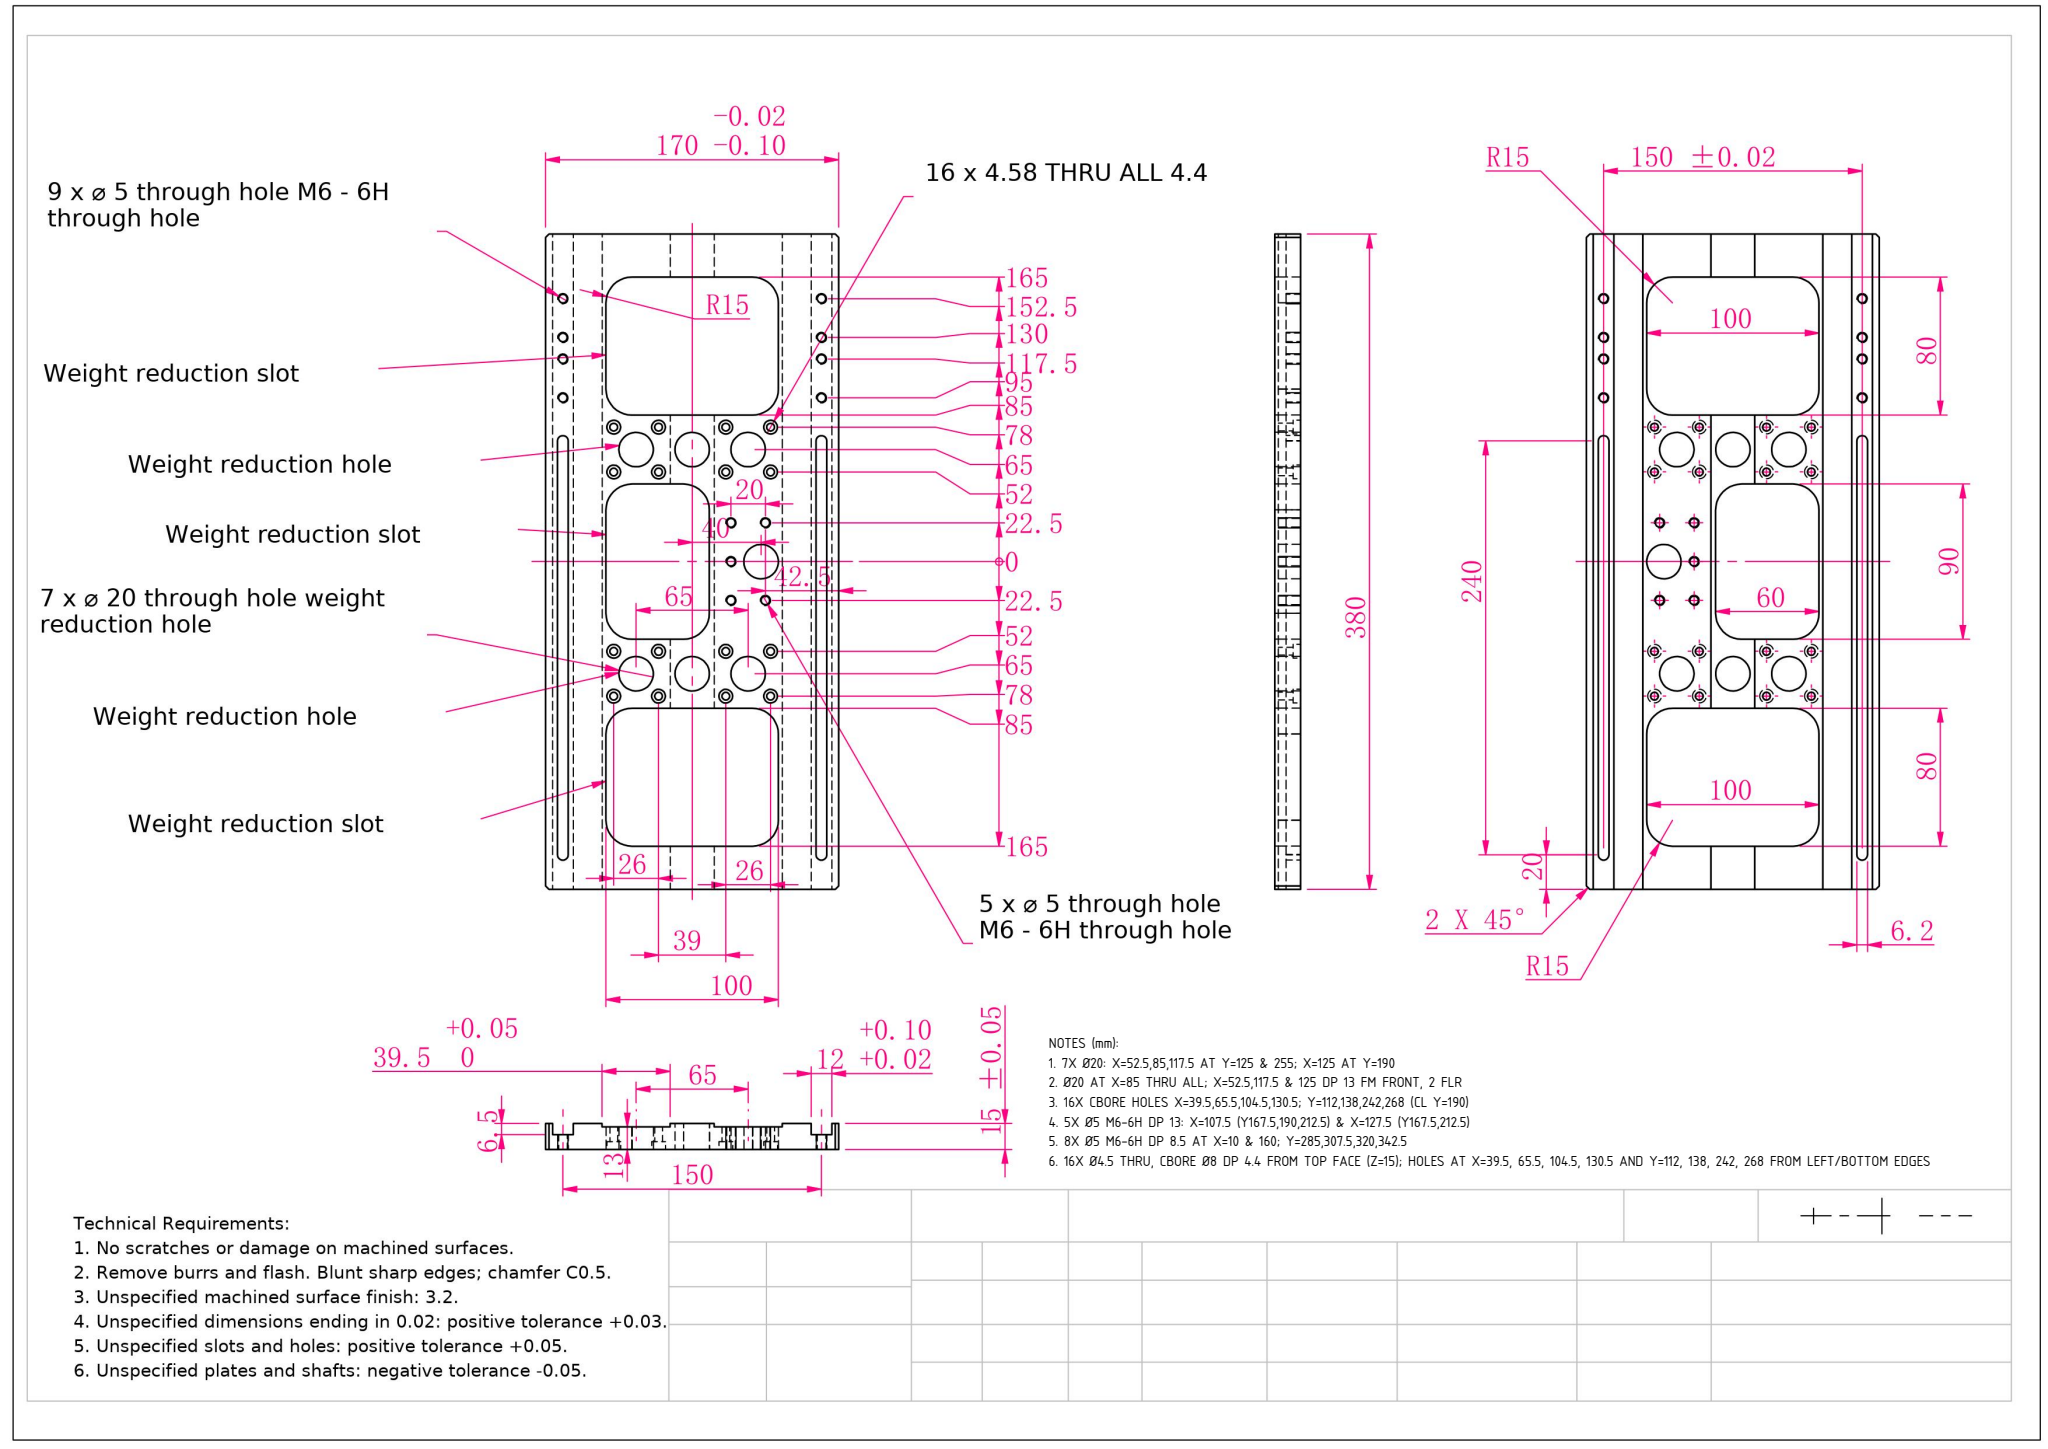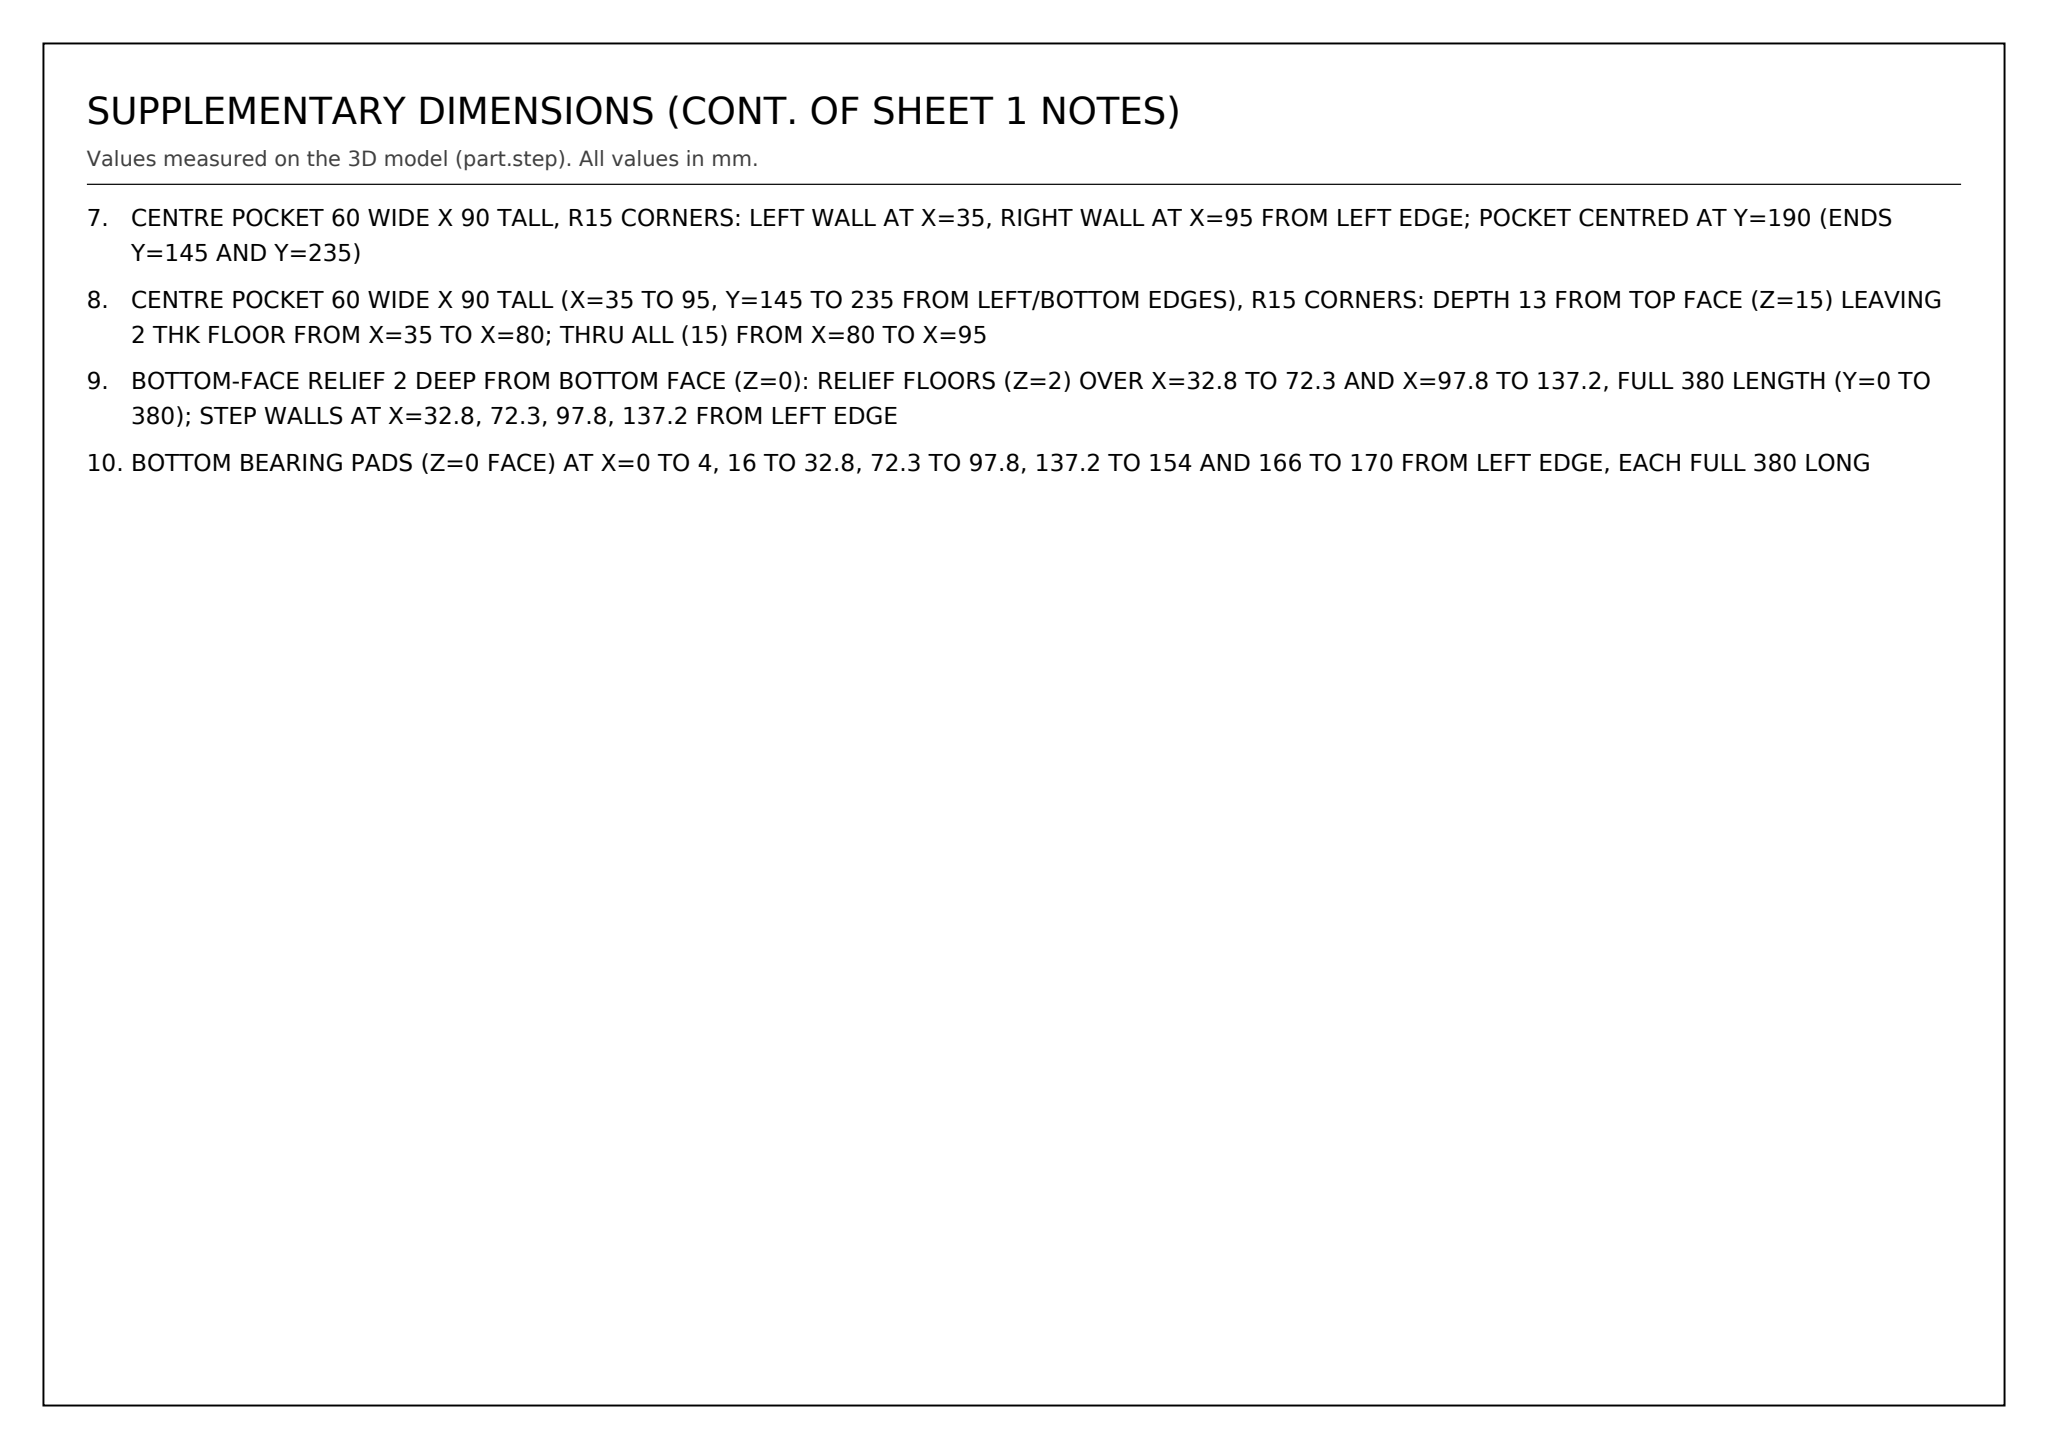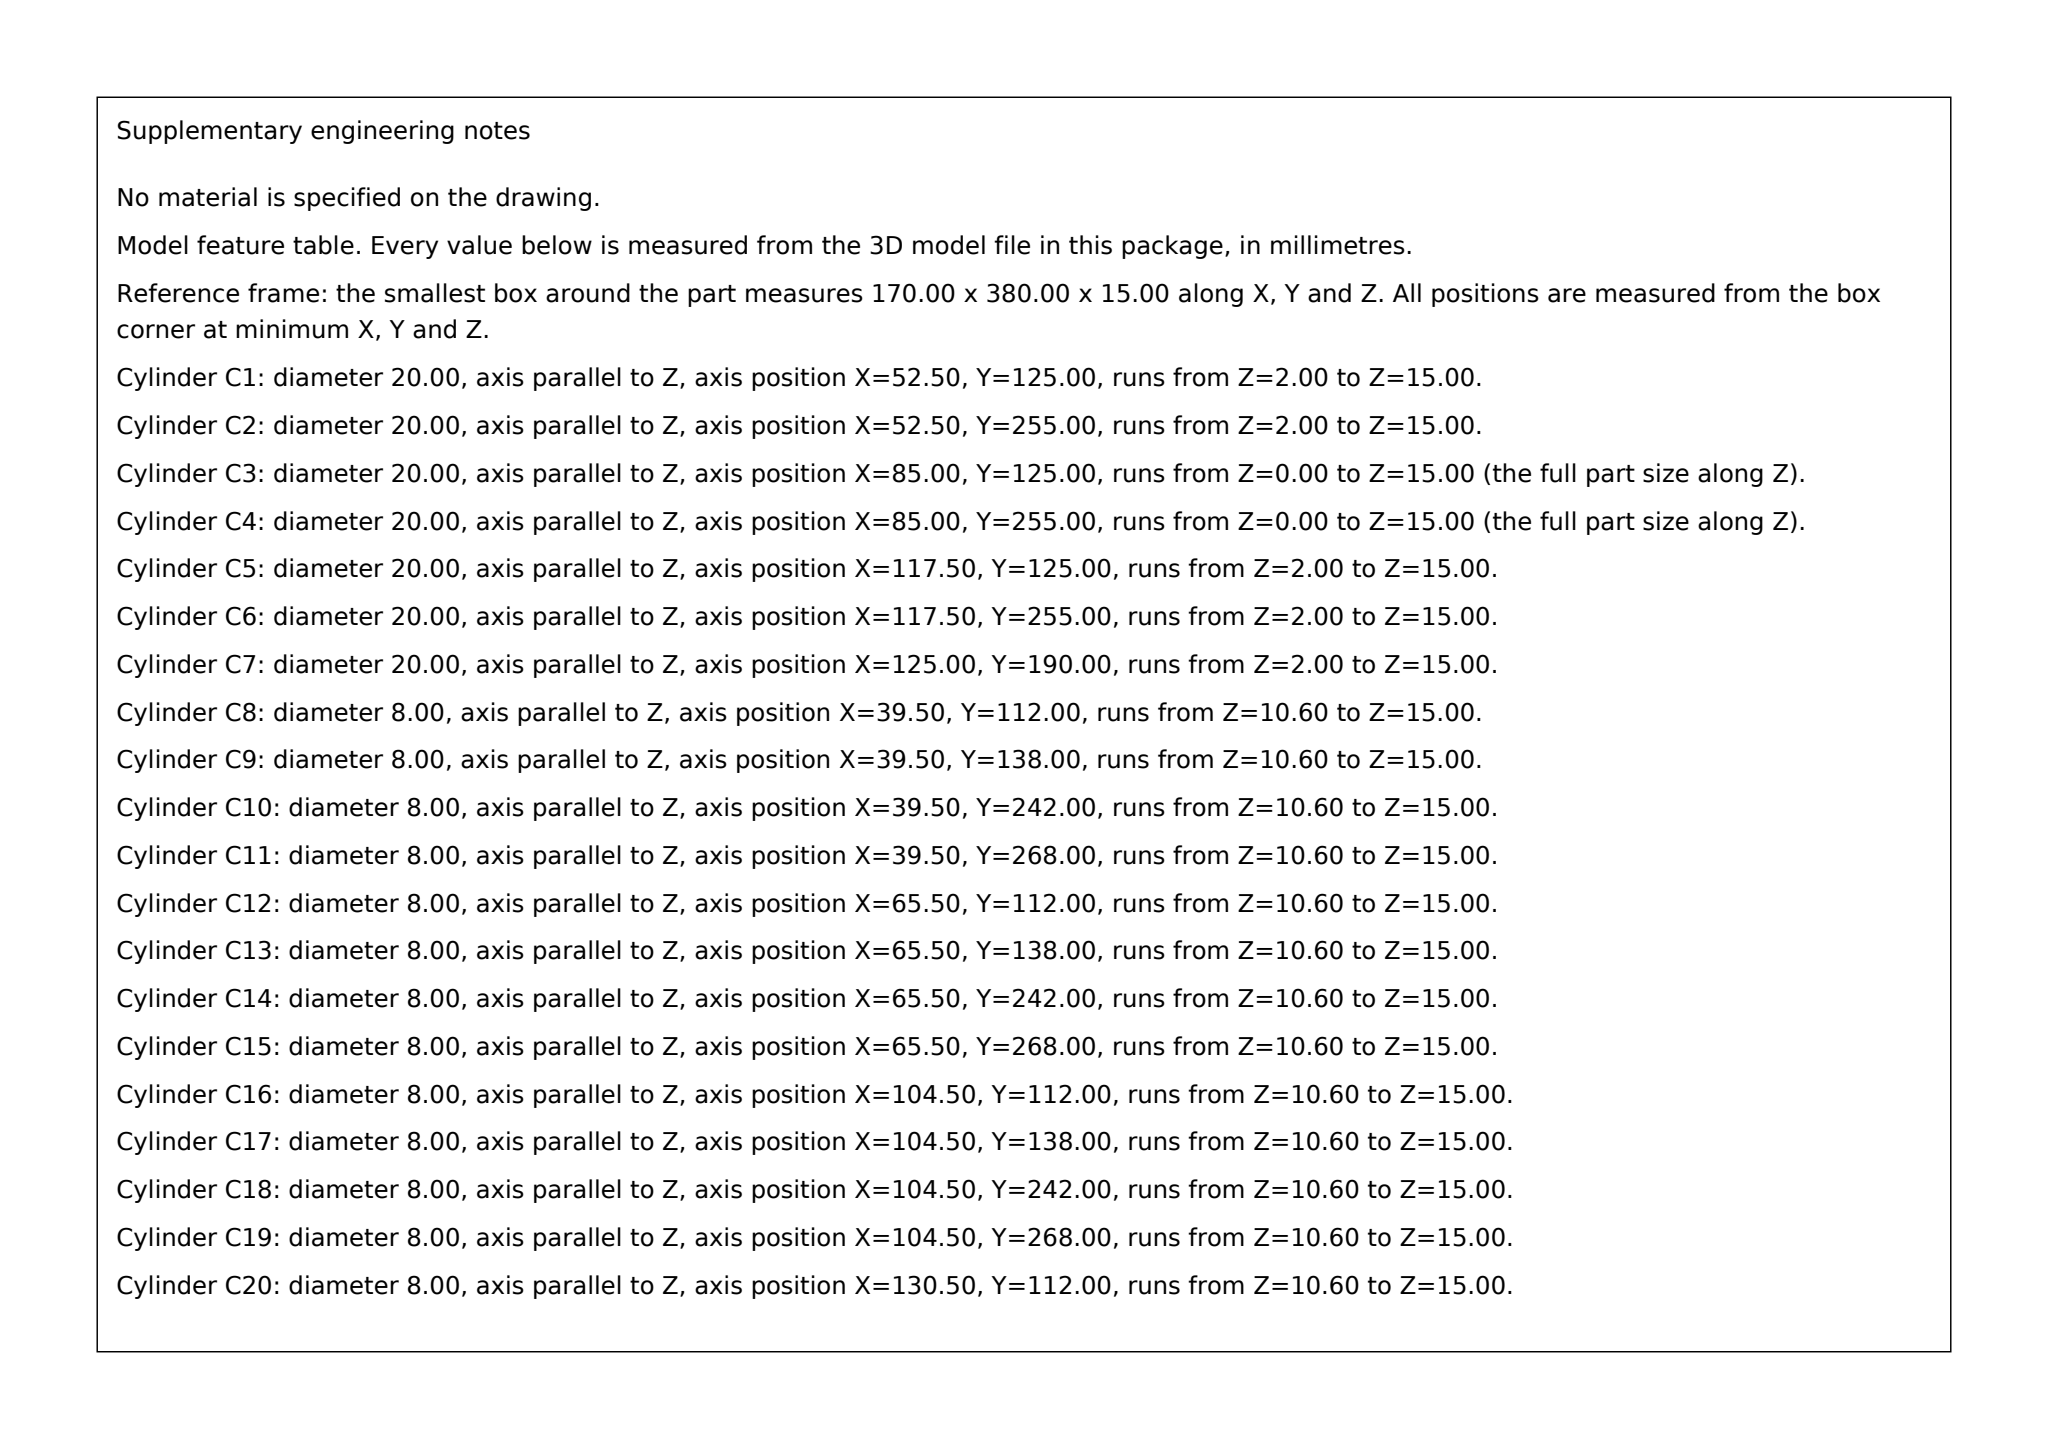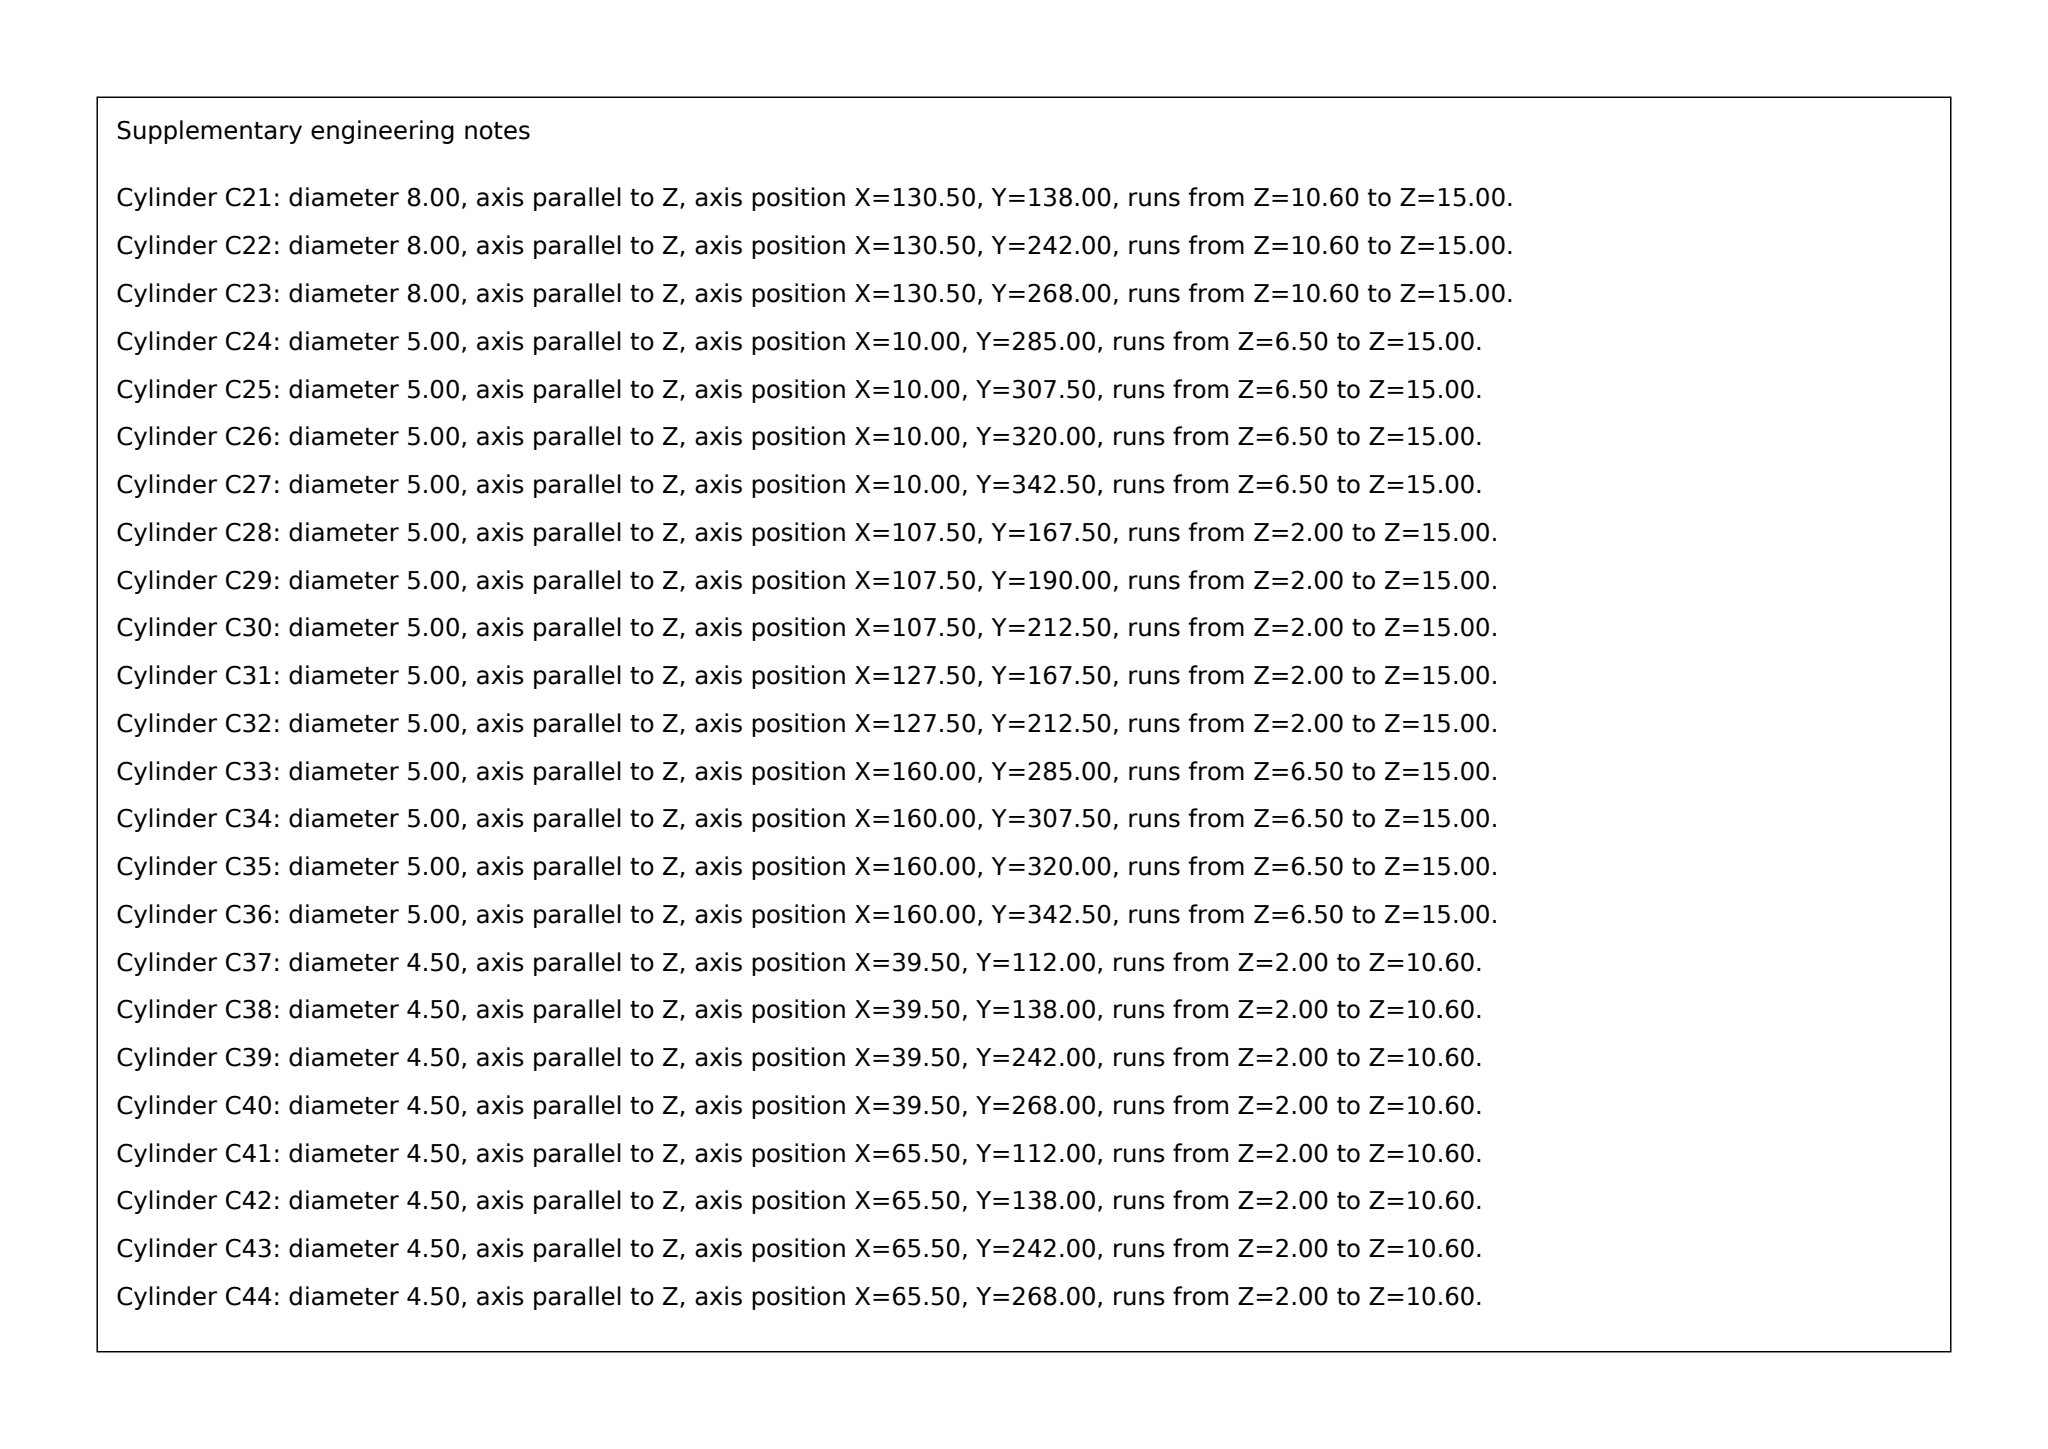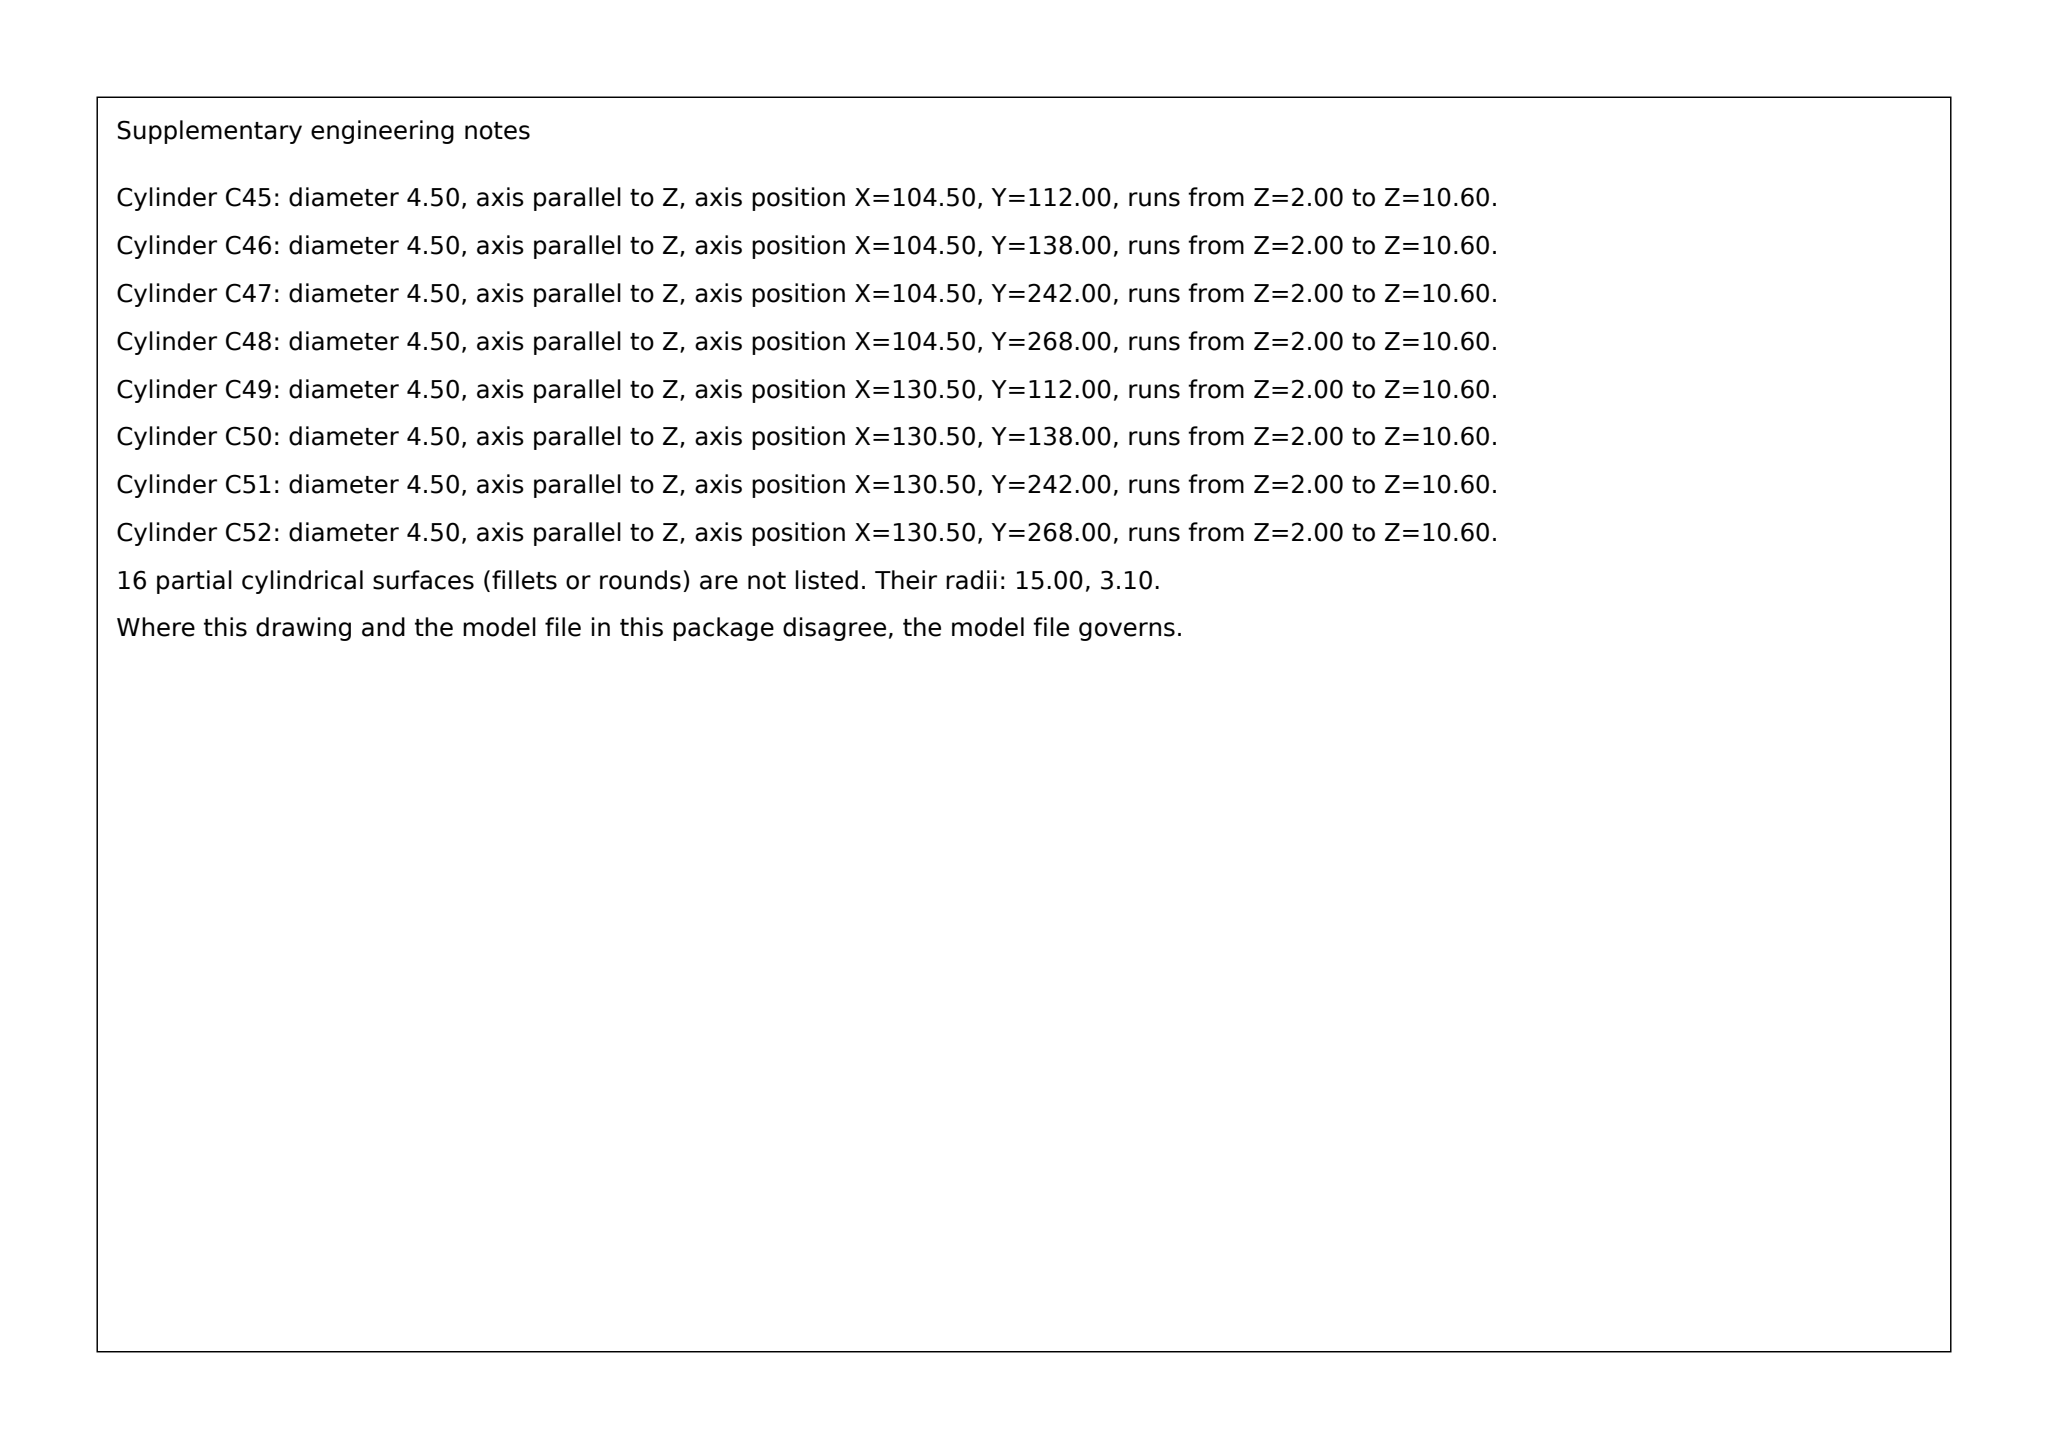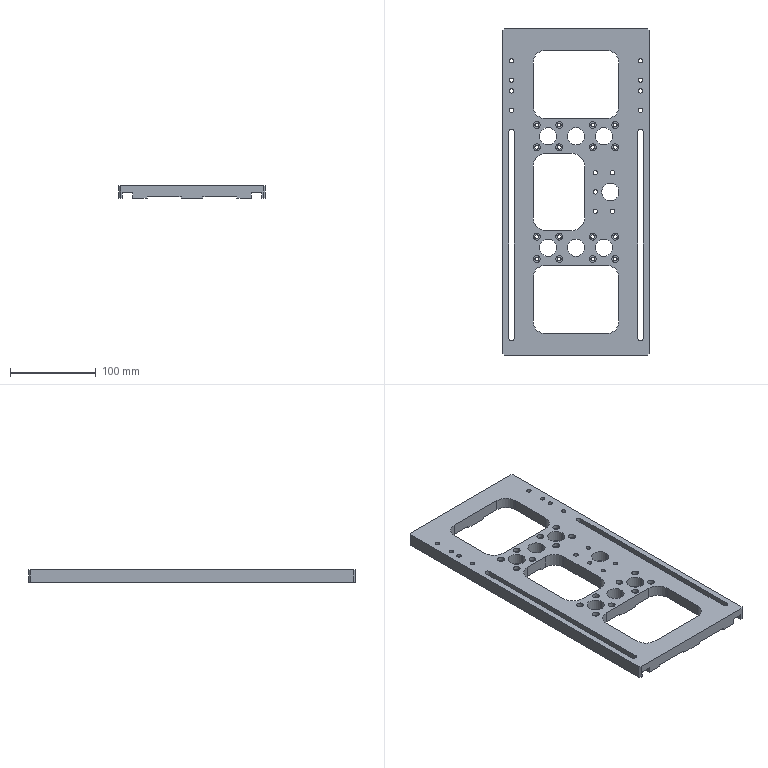Part | SolidWorks | mm | 1 solid | 185 faces | box 170 x 380 x 15 mm | volume 502838 mm3 | cylinder 120 | plane 65 | commonest cylinder face diameters 8 x32 4.5 x32 5 x26 20 x14 30 x12 6.2 x4
Drawing notes:
7X Ø20: X=52.5,85,117.5 AT Y=125 & 255; X=125 AT Y=190 | from the solid: Ø20 cyls at (52.5,125/255),(85,125/255),(117.5,125/255),(125,190)
Ø20 AT X=85 THRU ALL; X=52.5,117.5 & 125 DP 13 FM FRONT, 2 FLR | from the solid: Ø20 L=15 at (85,125)&(85,255); L=13 at (52.5,125/255),(117.5,125/255),(125,190); THK 15, z-plane 2.0
16X CBORE HOLES X=39.5,65.5,104.5,130.5; Y=112,138,242,268 (CL Y=190) | from the solid: Ø4.5/Ø8 holes at x=39.5,65.5,104.5,130.5 (26/39/26) and y=112,138,242,268 vs CL 190
5X Ø5 M6-6H DP 13: X=107.5 (Y167.5,190,212.5) & X=127.5 (Y167.5,212.5) | from the solid: Ø5 z-cyls L13 at x=107.5 (y167.5/190/212.5) and x=127.5 (y167.5/212.5); 20 apart, 22.5 fm CL
8X Ø5 M6-6H DP 8.5 AT X=10 & 160; Y=285,307.5,320,342.5 | from the solid: Ø5 L8.5 cyls at x=10 and x=160, y=285,307.5,320,342.5 = 4 per side, 8 total (not 9)
16X Ø4.5 THRU, CBORE Ø8 DP 4.4 FROM TOP FACE (Z=15); HOLES AT X=39.5, 65.5, 104.5, 130.5 AND Y=112, 138, 242, 268 FROM LEFT/BOTTOM EDGES | from the solid: cylinders: 16 bores dia 4.5 z from 2.0 to 10.6 and 16 coaxial bores dia 8.0 z from 10.6 to 15.0 at X=39.5,65.5,104.5,130.5 / Y=112,138,242,268; bbox_xyz z=15
CENTRE POCKET 60 WIDE X 90 TALL, R15 CORNERS: LEFT WALL AT X=35, RIGHT WALL AT X=95 FROM LEFT EDGE; POCKET CENTRED AT Y=190 (ENDS Y=145 AND Y=235) | from the solid: axis_planes x=35 and x=95 with y extent 160-220; axis_planes y=145 and y=235 with x extent 50-80; concave R15 (dia 30) corner arcs at (50,160),(50,220),(80,160),(80,220)
CENTRE POCKET 60 WIDE X 90 TALL (X=35 TO 95, Y=145 TO 235 FROM LEFT/BOTTOM EDGES), R15 CORNERS: DEPTH 13 FROM TOP FACE (Z=15) LEAVING 2 THK FLOOR FROM X=35 TO X=80; THRU ALL (15) FROM X=80 TO X=95 | from the solid: axis_planes x=35 y[160,220] z[2,15] and x=95 y[160,220] z[0,15]; concave R15 arcs at (50,160)/(50,220) z 2->15 and (80,160)/(80,220) z 0->15; bbox z=15
BOTTOM-FACE RELIEF 2 DEEP FROM BOTTOM FACE (Z=0): RELIEF FLOORS (Z=2) OVER X=32.8 TO 72.3 AND X=97.8 TO 137.2, FULL 380 LENGTH (Y=0 TO 380); STEP WALLS AT X=32.8, 72.3, 97.8, 137.2 FROM LEFT EDGE | from the solid: axis_planes x=32.8 / x=72.3 / x=97.7 / x=137.2 each with z extent [0.0,2.0] spanning y 0-380, plus z=0 pad faces listed only at x [0,4],[16,32.8],[72.3,97.8],[137.2,154],[166,170]
BOTTOM BEARING PADS (Z=0 FACE) AT X=0 TO 4, 16 TO 32.8, 72.3 TO 97.8, 137.2 TO 154 AND 166 TO 170 FROM LEFT EDGE, EACH FULL 380 LONG | from the solid: z=0 planes with extents x[0,4], x[16,32.8], x[72.3,97.8], x[137.2,154], x[166,170], y[0,380]
build123d program:
from build123d import *

# Parameters (mm, degrees)
SKETCH1_W                                       = 170
SKETCH1_H                                       = 380
BOSS_EXTRUDE1_DEPTH                             = 7.5
SKETCH2_W                                       = 39.5
SKETCH2_H                                       = 380
CUT_EXTRUDE1_DEPTH                              = 2
SKETCH7_W                                       = 100
SKETCH7_H                                       = 80
SKETCH7_W_2                                     = 60
SKETCH7_H_2                                     = 90
CUT_EXTRUDE4_DEPTH                              = 209.686
FILLET1_R                                       = 15
M6_TAPPED_HOLE1_D                               = 5
M4_HEX_SOCKET_HEAD_CAP_SCREW_CBORE1_D           = 4.5
M4_HEX_SOCKET_HEAD_CAP_SCREW_CBORE1_CBORE_D     = 8
M4_HEX_SOCKET_HEAD_CAP_SCREW_CBORE1_CBORE_DEPTH = 4.4
SKETCH12_W                                      = 12
SKETCH12_H                                      = 380
CUT_EXTRUDE5_DEPTH                              = 6.5
CUT_EXTRUDE6_DEPTH                              = 209.686
M6_TAPPED_HOLE2_D                               = 5
F_20_0_20_DIAMETER_HOLE1_D                      = 20
CHAMFER1_SIZE                                   = 2


with BuildPart() as part:
    # Sketch1 → Boss-Extrude1 (new, symmetric)
    with BuildSketch(Plane.XY):
        Rectangle(SKETCH1_W, SKETCH1_H)
    extrude(amount=BOSS_EXTRUDE1_DEPTH, both=True)

    # Sketch2 → Cut-Extrude1 (cut)
    with BuildSketch(Plane(origin=(0, 0, -7.5), x_dir=(-1, 0, 0), z_dir=(0, 0, -1))):
        with Locations((-32.5, 0)):
            Rectangle(SKETCH2_W, SKETCH2_H)
        with Locations((32.5, 0)):
            Rectangle(SKETCH2_W, SKETCH2_H)
    extrude(amount=-CUT_EXTRUDE1_DEPTH, mode=Mode.SUBTRACT)

    # Sketch7 → Cut-Extrude4 (cut, through all)
    with BuildSketch(Plane.XY.offset(7.5)):
        with Locations((0, -125)):
            Rectangle(SKETCH7_W, SKETCH7_H)
        with Locations((-20, 0)):
            Rectangle(SKETCH7_W_2, SKETCH7_H_2)
        with Locations((0, 125)):
            Rectangle(SKETCH7_W, SKETCH7_H)
    extrude(amount=-CUT_EXTRUDE4_DEPTH, mode=Mode.SUBTRACT)

    # Fillet1
    fillet1_edges = [part.edges().sort_by_distance(p)[0] for p in [
        (-50, -85, 1),
        (50, -165, 1),
        (-50, -165, 1),
        (50, -85, 1),
        (-50, 45, 1),
        (10, -45, 0),
        (-50, -45, 1),
        (10, 45, 0),
        (-50, 165, 1),
        (50, 85, 1),
        (-50, 85, 1),
        (50, 165, 1),
    ]]
    fillet(fillet1_edges, radius=FILLET1_R)

    # M6 Tapped Hole1 (through all)
    with Locations(Plane(origin=(0, 0, -7.5), x_dir=(-1, 0, 0), z_dir=(0, 0, -1))):
        with Locations((-22.5, 22.5), (-42.5, 22.5), (-42.5, -22.5), (-22.5, -22.5), (-22.5, 0)):
            Hole(M6_TAPPED_HOLE1_D / 2)

    # M4 Hex Socket Head Cap Screw CBORE1 (through all)
    with Locations(Plane.XY.offset(7.5)):
        with Locations((45.5, -78), (45.5, -52), (19.5, -52), (19.5, -78), (-19.5, -52), (-19.5, -78), (-45.5, -78), (-45.5, -52), (-45.5, 52), (-45.5, 78), (-19.5, 78), (-19.5, 52), (19.5, 78), (19.5, 52), (45.5, 52), (45.5, 78)):
            CounterBoreHole(M4_HEX_SOCKET_HEAD_CAP_SCREW_CBORE1_D / 2, M4_HEX_SOCKET_HEAD_CAP_SCREW_CBORE1_CBORE_D / 2, M4_HEX_SOCKET_HEAD_CAP_SCREW_CBORE1_CBORE_DEPTH)

    # Sketch12 → Cut-Extrude5 (cut)
    with BuildSketch(Plane(origin=(0, 0, -7.5), x_dir=(-1, 0, 0), z_dir=(0, 0, -1))):
        with Locations((-75, 0)):
            Rectangle(SKETCH12_W, SKETCH12_H)
        with Locations((75, 0)):
            Rectangle(SKETCH12_W, SKETCH12_H)
    extrude(amount=-CUT_EXTRUDE5_DEPTH, mode=Mode.SUBTRACT)

    # Sketch13 → Cut-Extrude6 (cut, through all)
    with BuildSketch(Plane.XY.offset(7.5)):
        with BuildLine():
            Line((78.1, 70), (78.1, -170))
            ThreePointArc((78.1, -170), (75, -173.1), (71.9, -170))
            Line((71.9, -170), (71.9, 70))
            ThreePointArc((71.9, 70), (75, 73.1), (78.1, 70))
        make_face()
        with BuildLine():
            Line((-78.1, 70), (-78.1, -170))
            ThreePointArc((-78.1, -170), (-75, -173.1), (-71.9, -170))
            Line((-71.9, -170), (-71.9, 70))
            ThreePointArc((-71.9, 70), (-75, 73.1), (-78.1, 70))
        make_face()
    extrude(amount=-CUT_EXTRUDE6_DEPTH, mode=Mode.SUBTRACT)

    # M6 Tapped Hole2 (through all)
    with Locations(Plane.XY.offset(7.5)):
        with Locations((75, 95), (75, 117.5), (75, 130), (75, 152.5), (186.536, 308.279), (-75, 152.5), (-75, 130), (-75, 117.5), (-75, 95)):
            Hole(M6_TAPPED_HOLE2_D / 2)

    # 20.0 _20_ Diameter Hole1 (through all)
    with Locations(Plane(origin=(0, 0, -7.5), x_dir=(-1, 0, 0), z_dir=(0, 0, -1))):
        with Locations((0, -65), (-32.5, -65), (32.5, -65), (32.5, 65), (-32.5, 65), (0, 65), (-40, 0)):
            Hole(F_20_0_20_DIAMETER_HOLE1_D / 2)

    # Chamfer1
    chamfer1_edges = [part.edges().sort_by_distance(p)[0] for p in [
        (85, -190, 0),
        (-85, -190, 0),
        (-85, 190, 0),
        (85, 190, 0),
    ]]
    chamfer(chamfer1_edges, length=CHAMFER1_SIZE)


solid = part.part